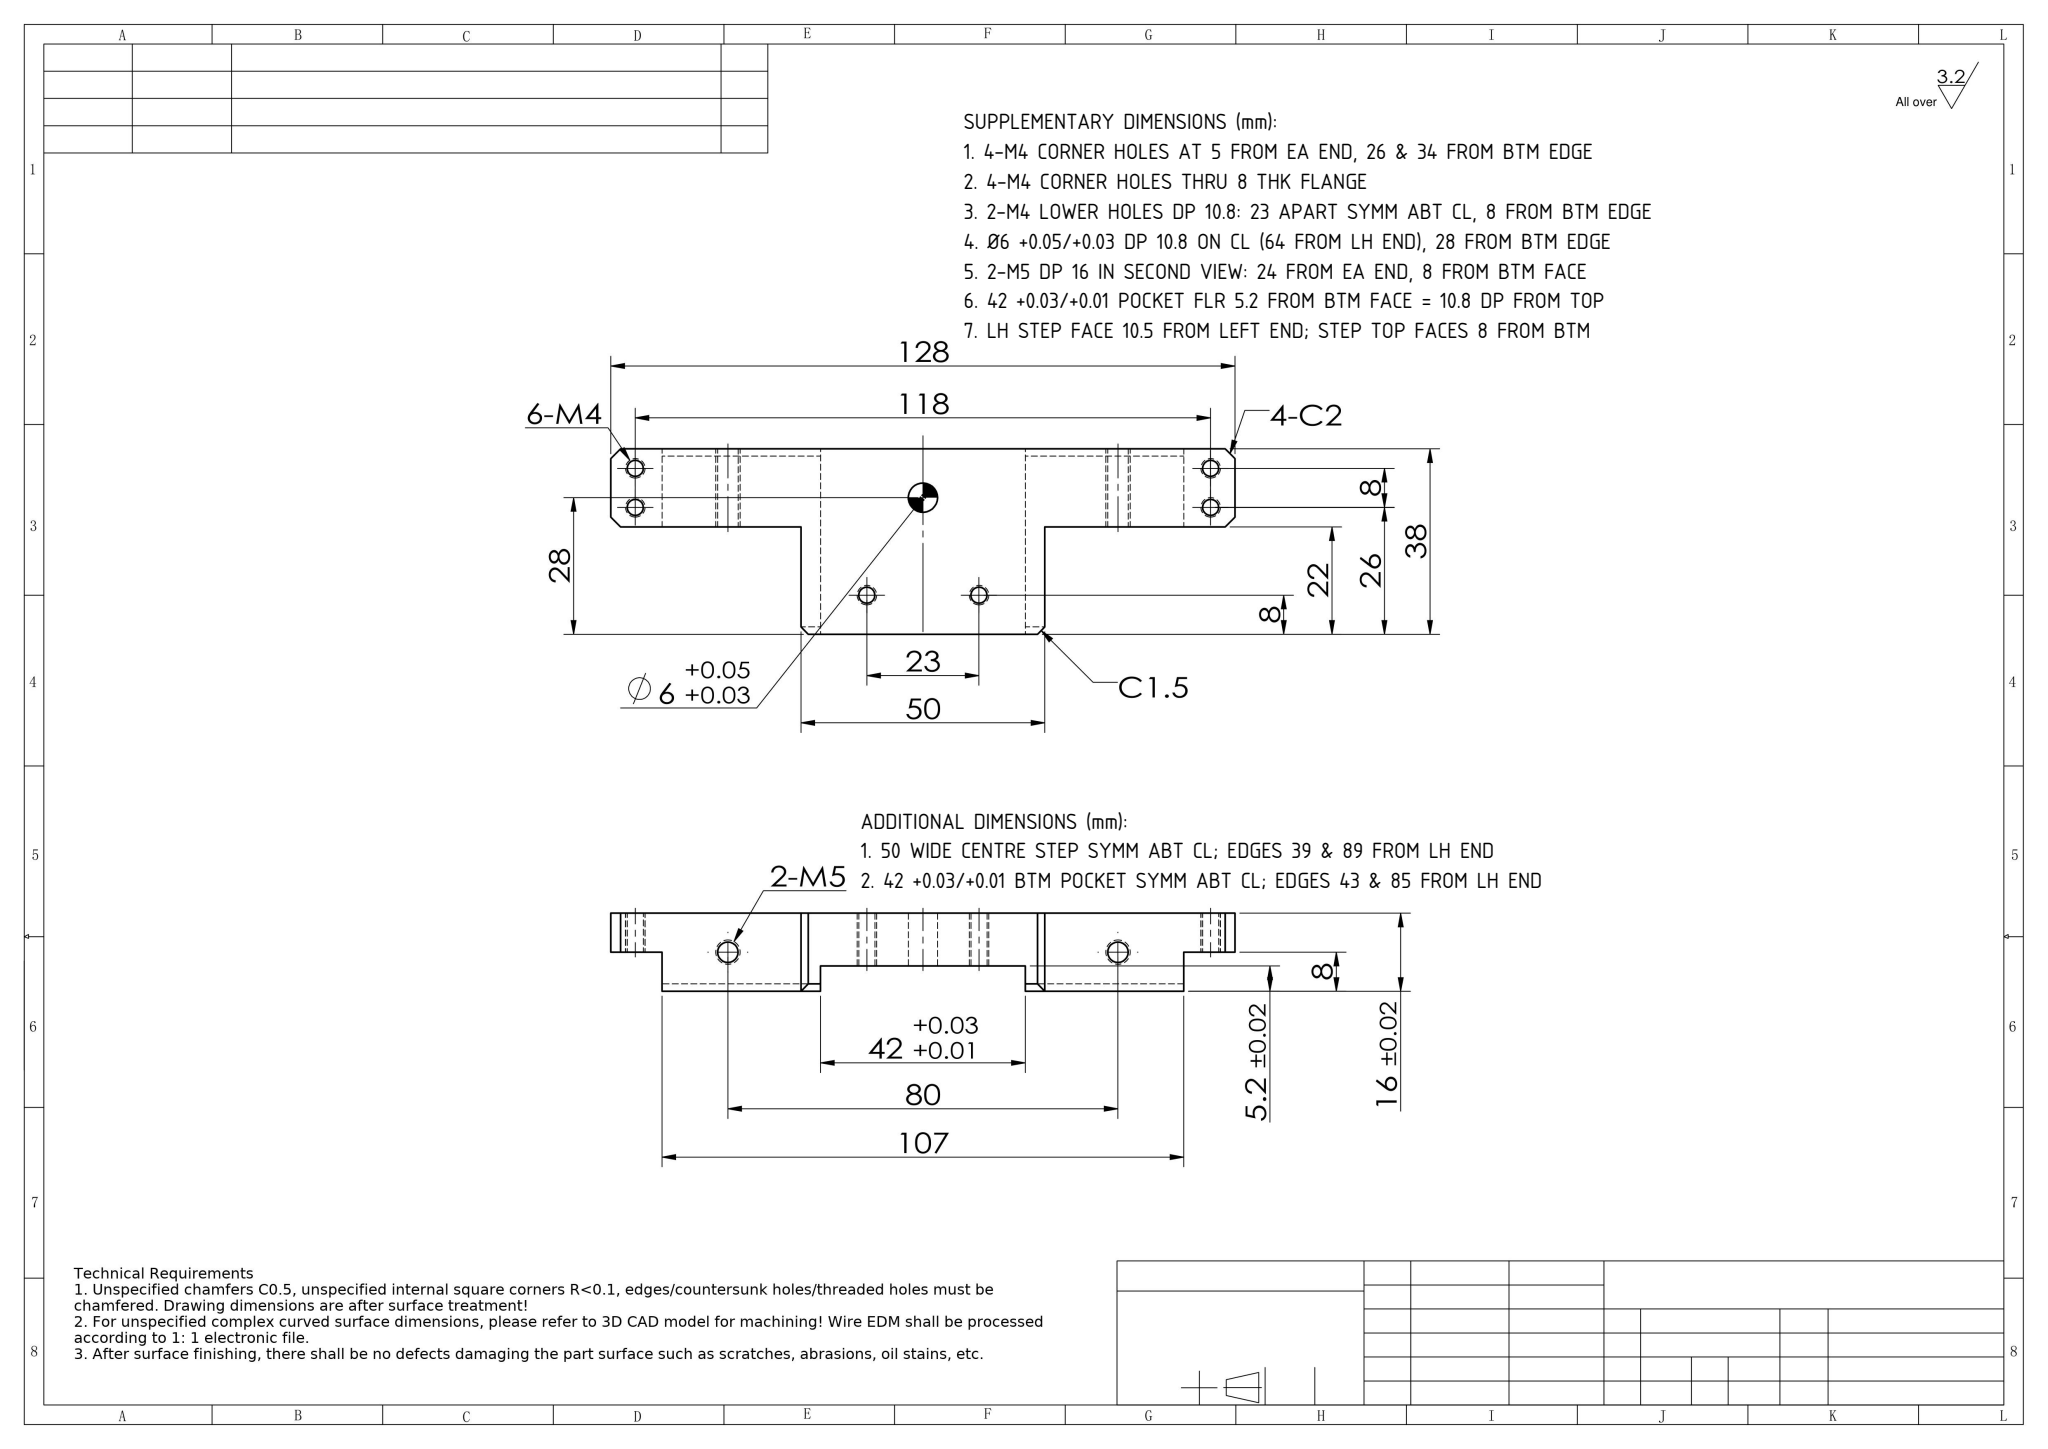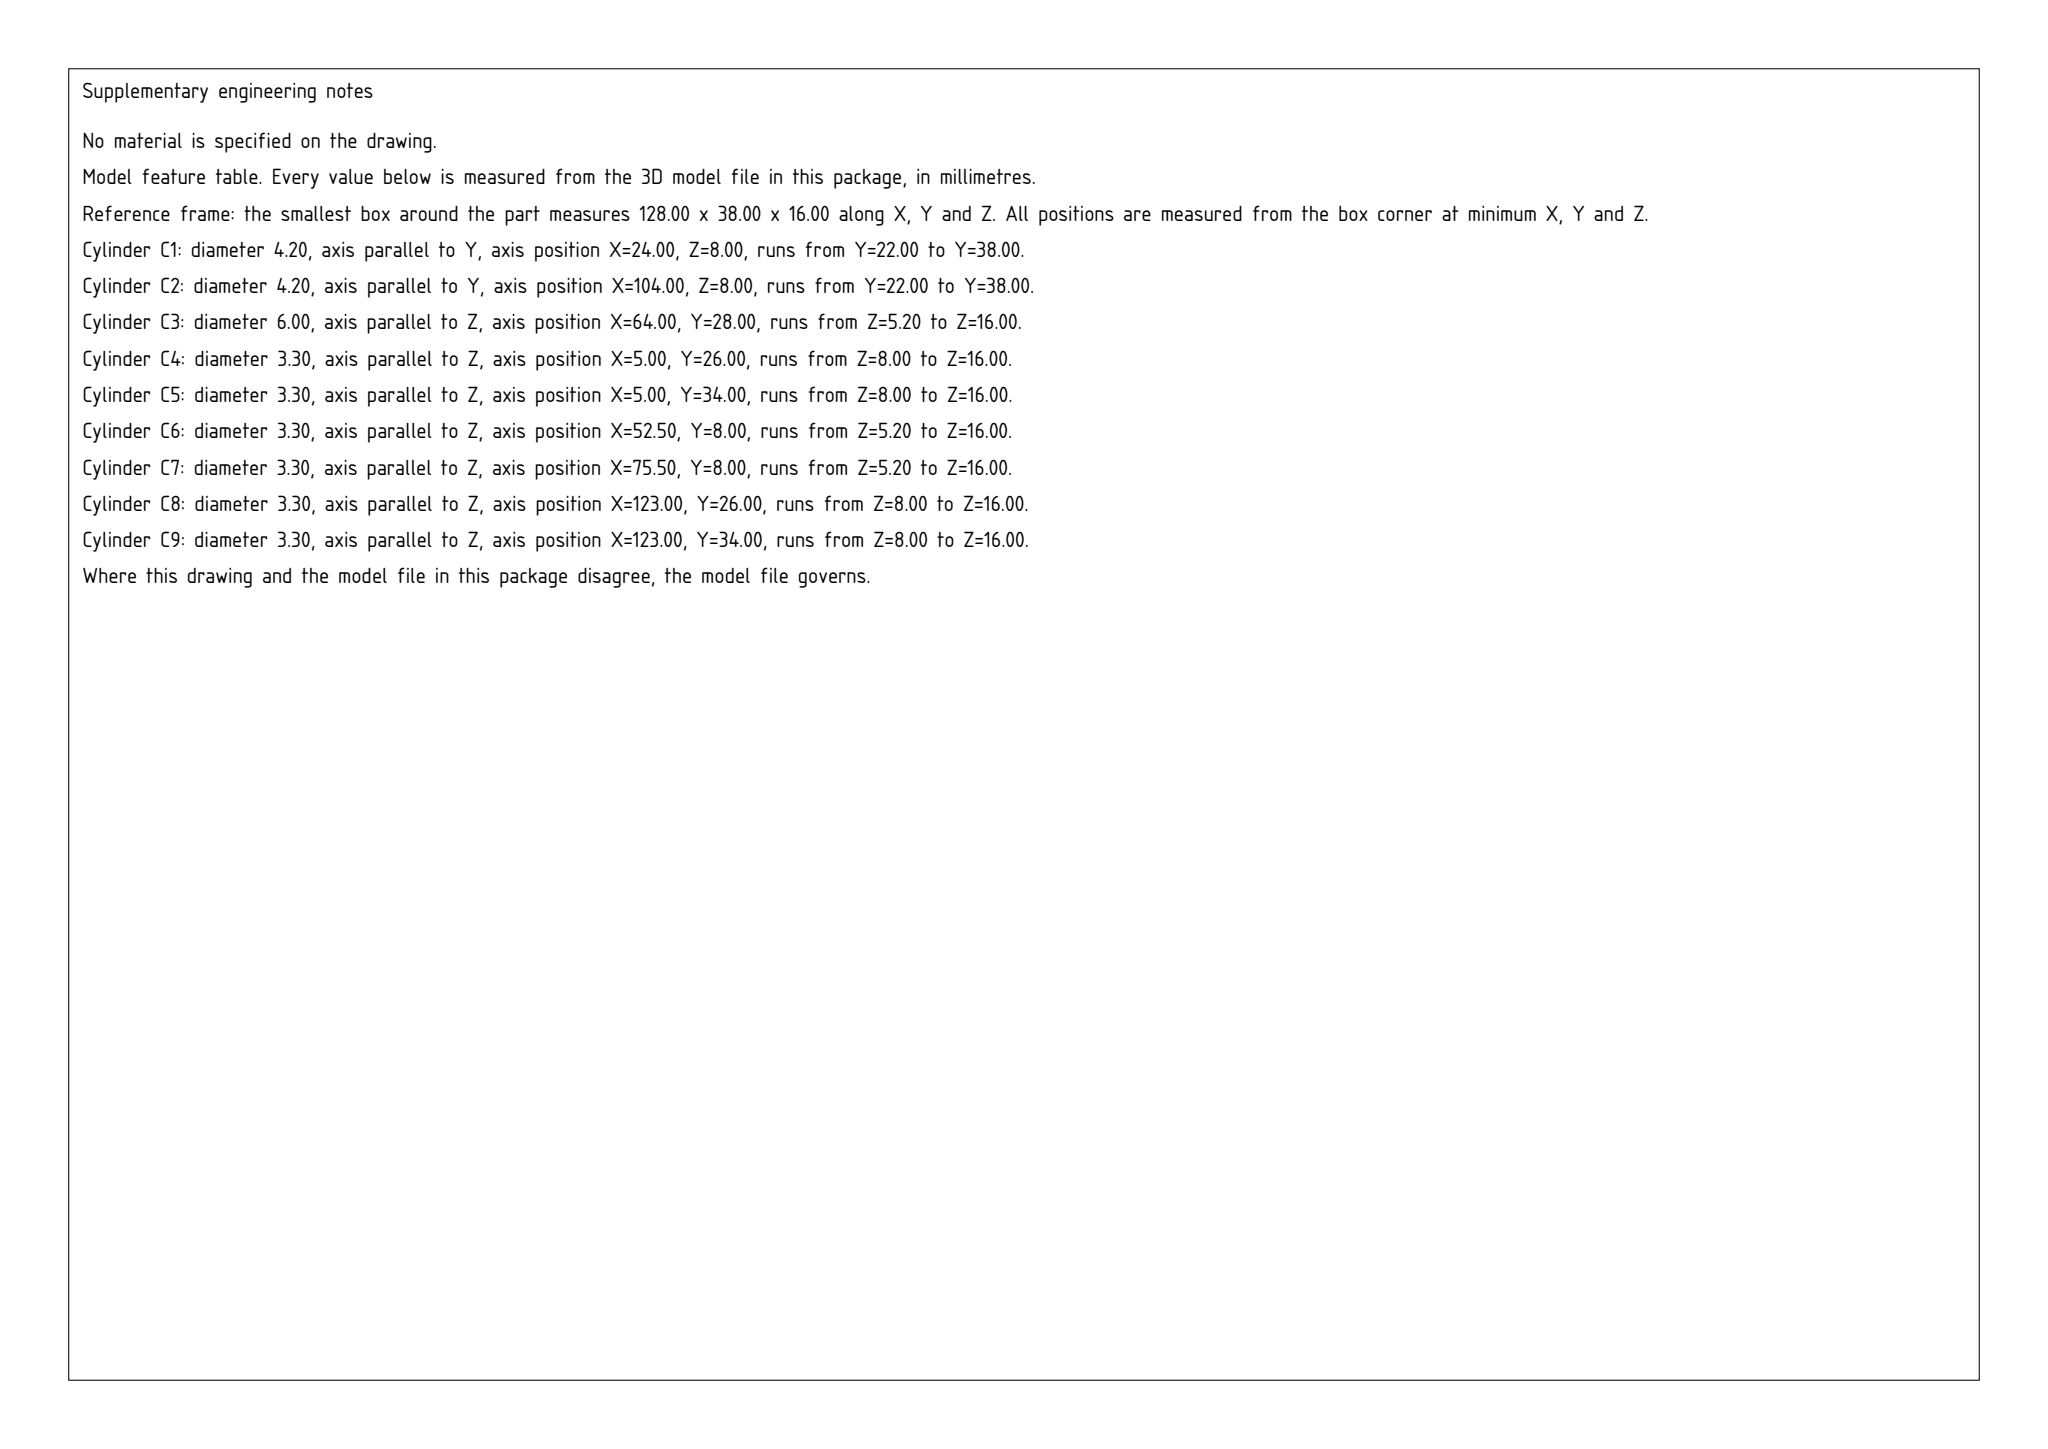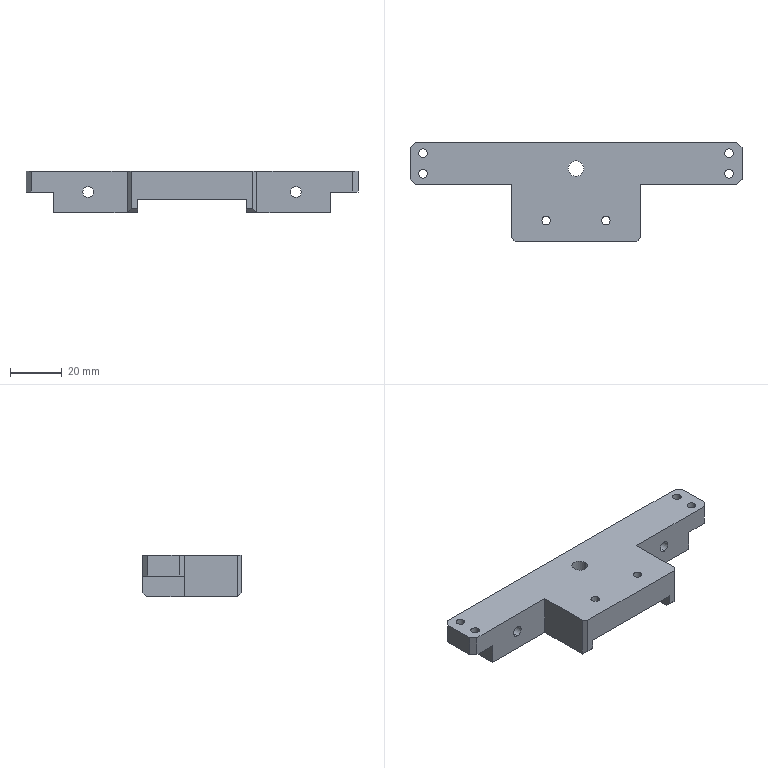Part | SolidWorks | mm | 1 solid | 46 faces | box 128 x 38 x 16 mm | volume 37994 mm3 | plane 28 | cylinder 18 | commonest cylinder face diameters 3.3 x12 4.2 x4 6 x2
build123d program:
from build123d import *

# Parameters (mm, degrees)
BOSS_EXTRUDE1_DEPTH        = 16
SKETCH2_W                  = 42
SKETCH2_H                  = 5.2
CUT_EXTRUDE1_DEPTH         = 77.131
M4_TAPPED_HOLE1_D          = 3.3
SIZE_MM_DOWEL_PIN_HOLE_1_D = 6
SKETCH12_W                 = 10.5
SKETCH12_H                 = 16
CUT_EXTRUDE2_DEPTH         = 8
M5_TAPPED_HOLE1_D          = 4.2
CHAMFER1_SIZE              = 2
CHAMFER2_SIZE              = 1.5


with BuildPart() as part:
    # Sketch1 → Boss-Extrude1 (new body)
    with BuildSketch(Plane.XY):
        Polygon((-64, 3), (-25, 3), (-25, -19), (25, -19), (25, 3), (64, 3), (64, 19), (-64, 19), align=None)
    extrude(amount=BOSS_EXTRUDE1_DEPTH)

    # Sketch2 → Cut-Extrude1 (cut, through all)
    with BuildSketch(Plane(origin=(0, 19, 0), x_dir=(1, 0, 0), z_dir=(0, 1, 0))):
        with Locations((0, -2.6)):
            Rectangle(SKETCH2_W, SKETCH2_H)
    extrude(amount=-CUT_EXTRUDE1_DEPTH, mode=Mode.SUBTRACT)

    # M4 Tapped Hole1 (through all)
    with Locations(Plane.XY.offset(16)):
        with Locations((59, 15), (59, 7), (11.5, -11), (-11.5, -11), (-59, 15), (-59, 7)):
            Hole(M4_TAPPED_HOLE1_D / 2)

    # Size mm Dowel Pin Hole 1 (through all)
    with Locations(Plane.XY.offset(16)):
        with Locations((0, 9)):
            Hole(SIZE_MM_DOWEL_PIN_HOLE_1_D / 2)

    # Sketch12 → Cut-Extrude2 (cut)
    with BuildSketch(Plane(origin=(0, 0, 0), x_dir=(-1, 0, 0), z_dir=(0, 0, -1))):
        with Locations((58.75, 11)):
            Rectangle(SKETCH12_W, SKETCH12_H)
        with Locations((-58.75, 11)):
            Rectangle(SKETCH12_W, SKETCH12_H)
    extrude(amount=-CUT_EXTRUDE2_DEPTH, mode=Mode.SUBTRACT)

    # M5 Tapped Hole1 (through all)
    with Locations(Plane(origin=(0, 19, 0), x_dir=(1, 0, 0), z_dir=(0, 1, 0))):
        with Locations((-40, -8), (40, -8)):
            Hole(M5_TAPPED_HOLE1_D / 2)

    # Chamfer1
    chamfer1_edges = [part.edges().sort_by_distance(p)[0] for p in [
        (-64, 19, 12),
        (64, 19, 12),
        (64, 3, 12),
        (-64, 3, 12),
    ]]
    chamfer(chamfer1_edges, length=CHAMFER1_SIZE)

    # Chamfer2
    chamfer2_edges = [part.edges().sort_by_distance(p)[0] for p in [
        (25, -19, 8),
        (-25, -19, 8),
        (-37.25, 19, 0),
        (23, -19, 0),
        (-23, -19, 0),
        (37.25, 19, 0),
    ]]
    chamfer(chamfer2_edges, length=CHAMFER2_SIZE)


solid = part.part